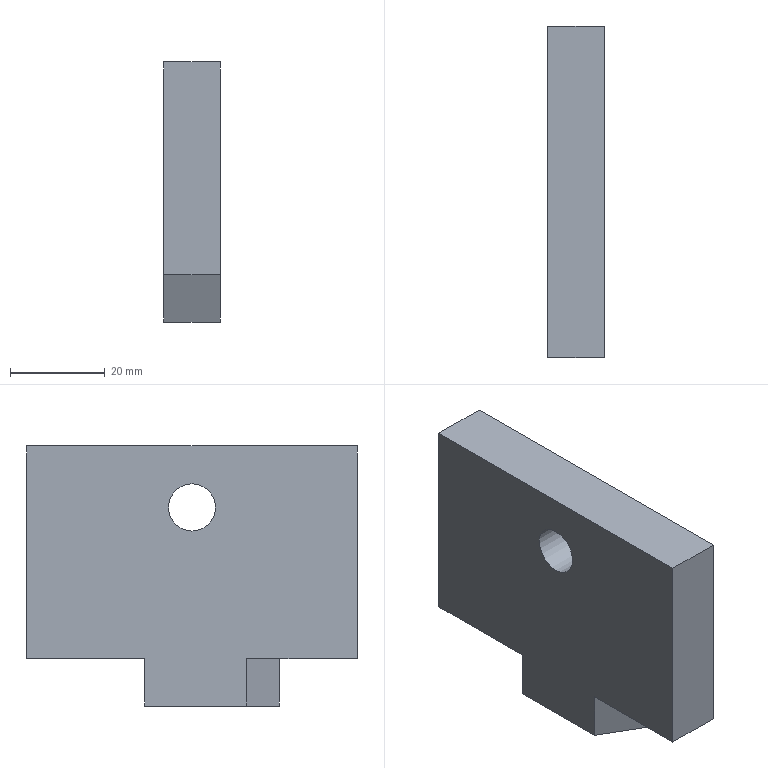Component | NX | SUPPORT_PLATE | 1 solid | 17 faces | volume 39295 mm3 | plane 10 | cone 4 | cylinder 3 | commonest cylinder face diameters 4.826 x2 10 x1